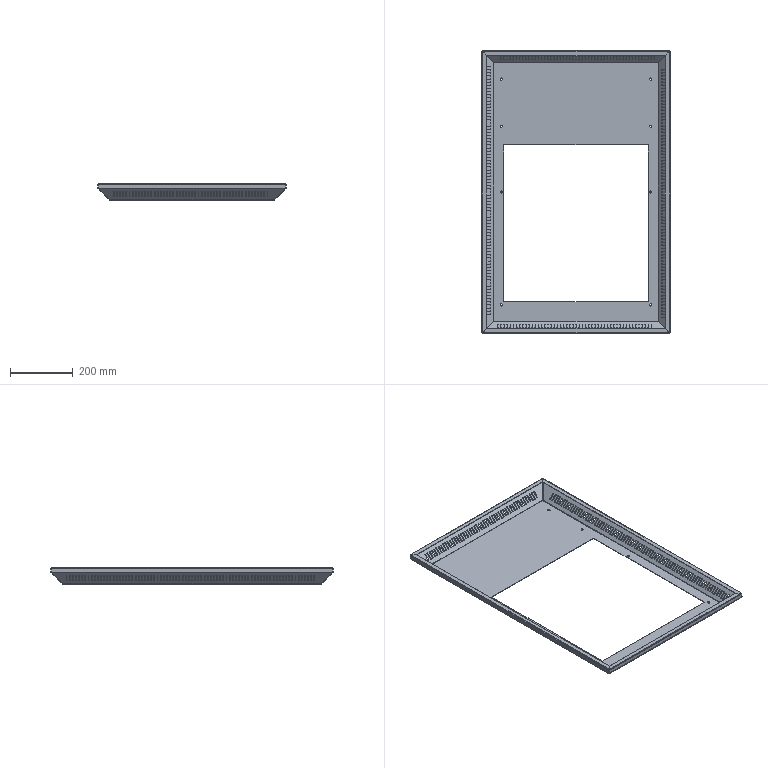Component | SolidWorks | TopCover-1 | 1 solid | 1422 faces | volume 620197 mm3 | cylinder 820 | plane 578 | spline 24 | commonest cylinder face diameters 3 x780 7 x16 2 x12 5 x12